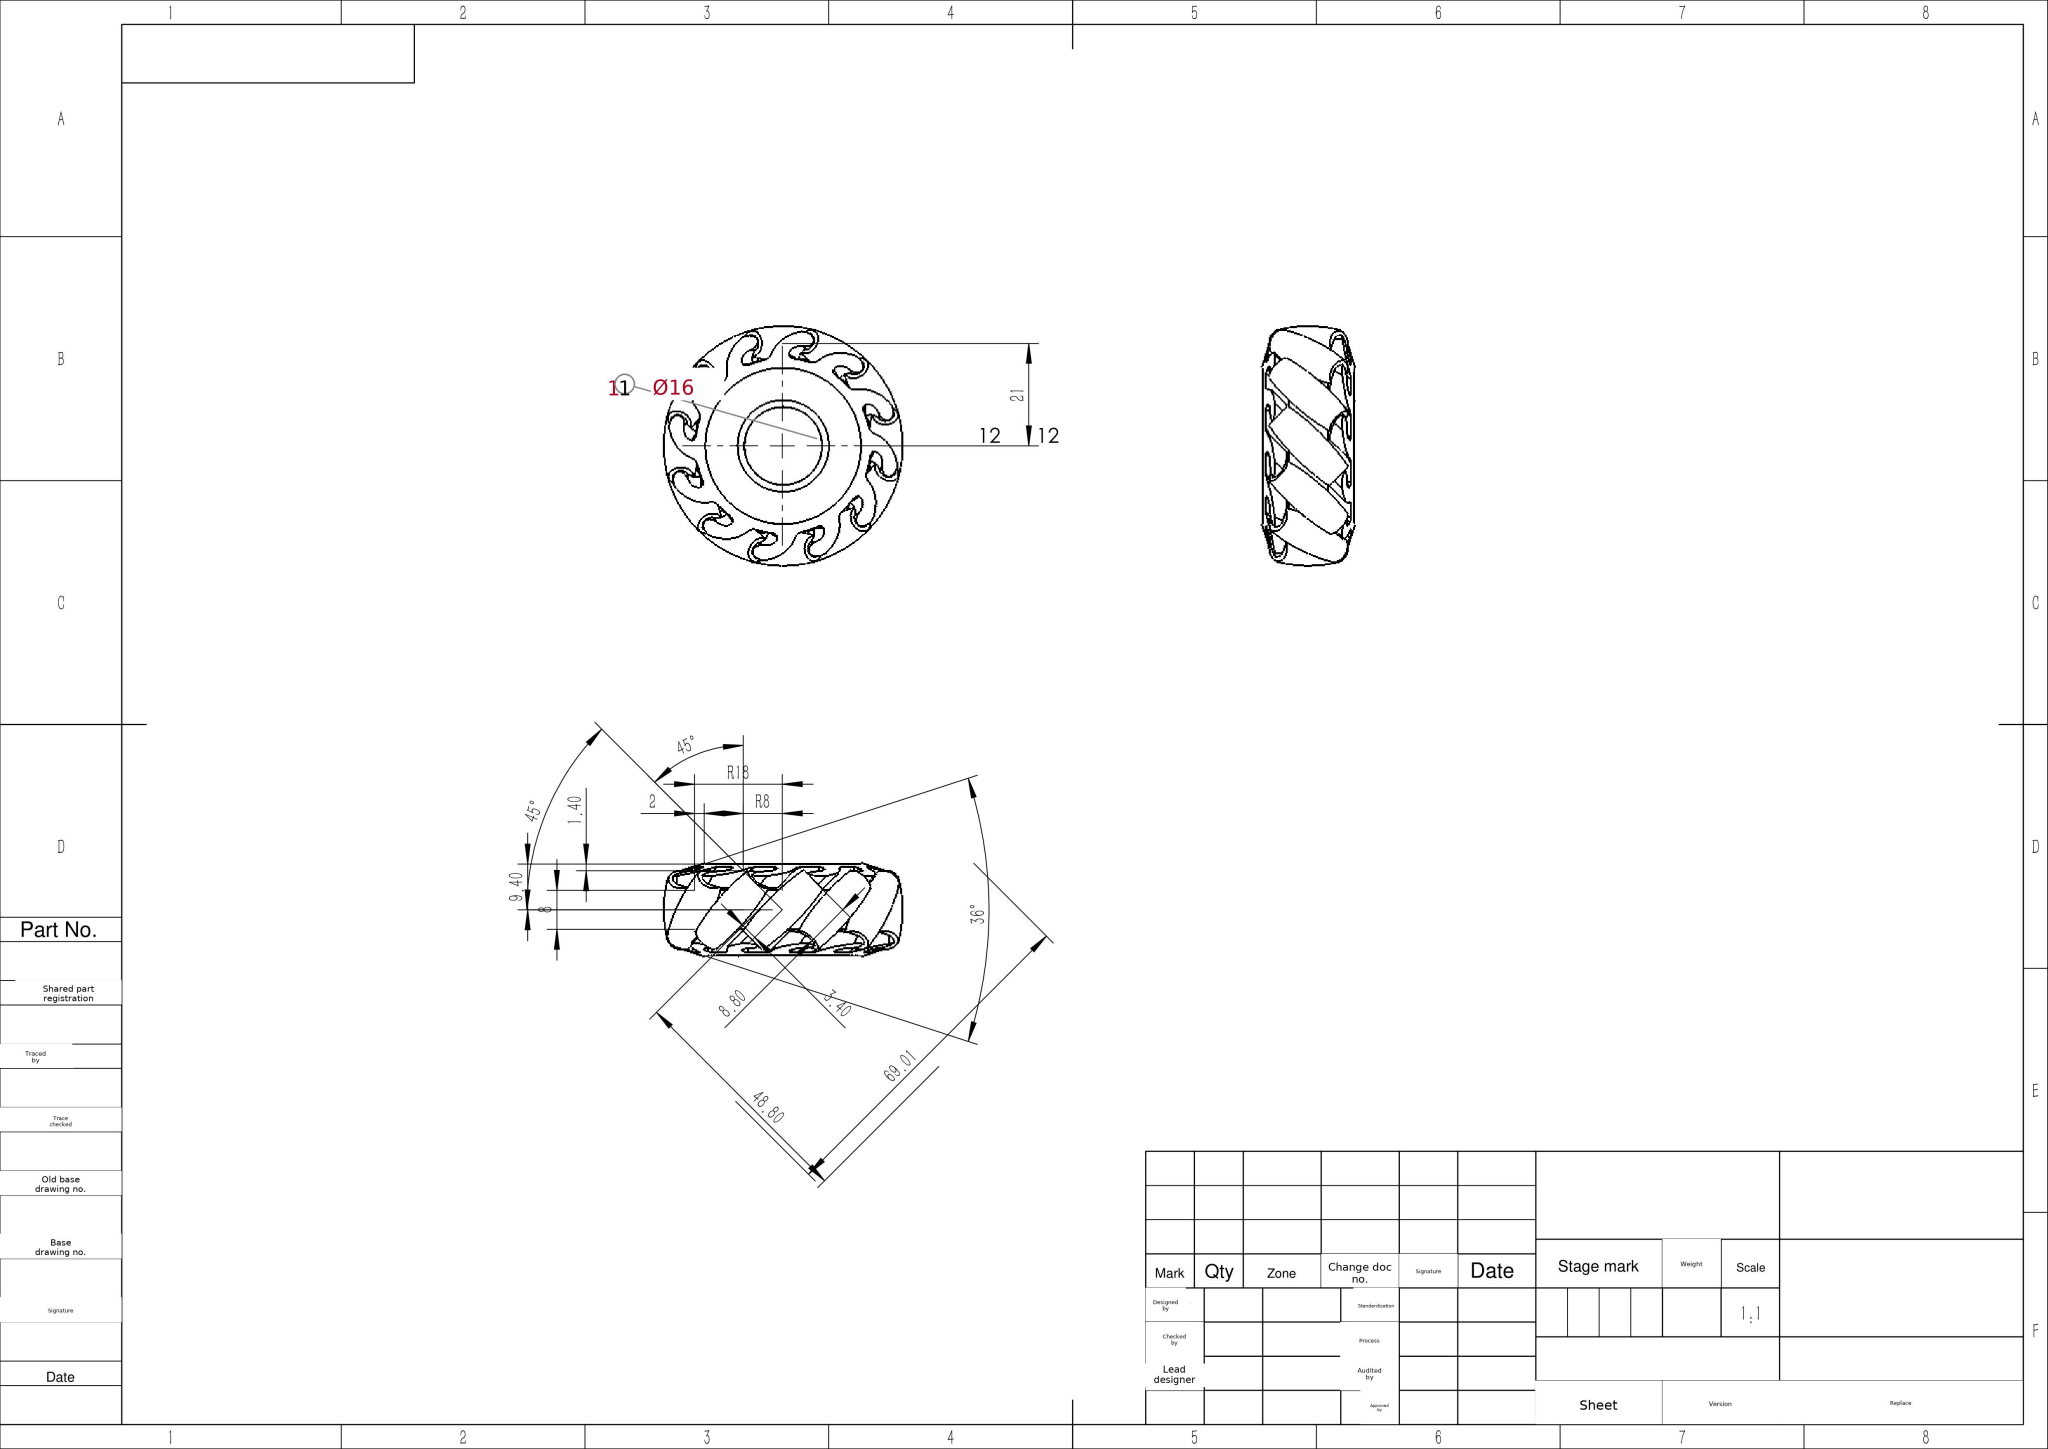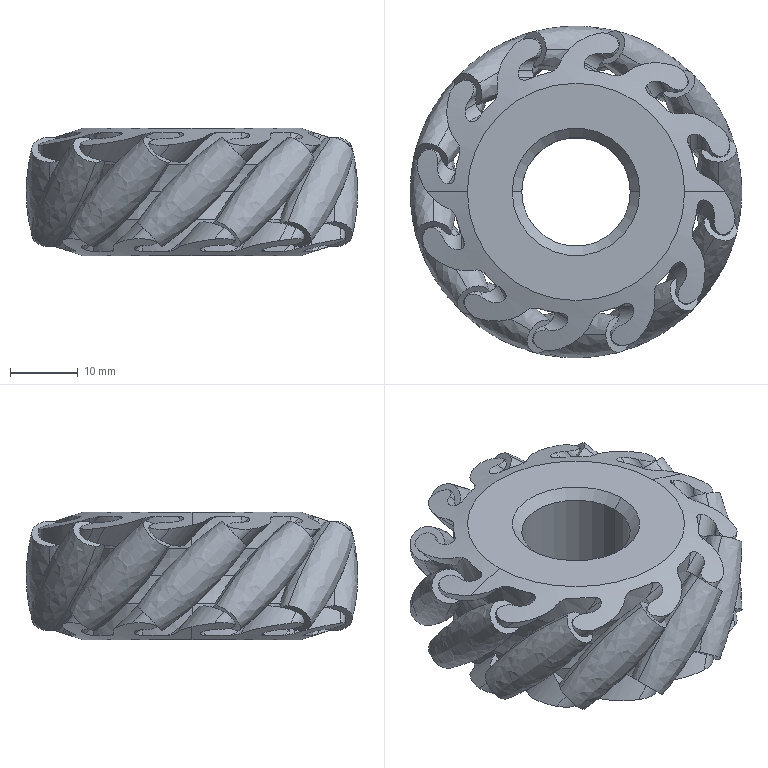Part | SolidWorks | mm | 1 solid | 252 faces | box 48.78 x 48.77 x 18.8 mm | volume 22534 mm3 | cylinder 166 | plane 50 | spline 24 | cone 8 | torus 4 | commonest cylinder face diameters 4 x68 3.2 x36 16 x34 1.6 x24 36 x4